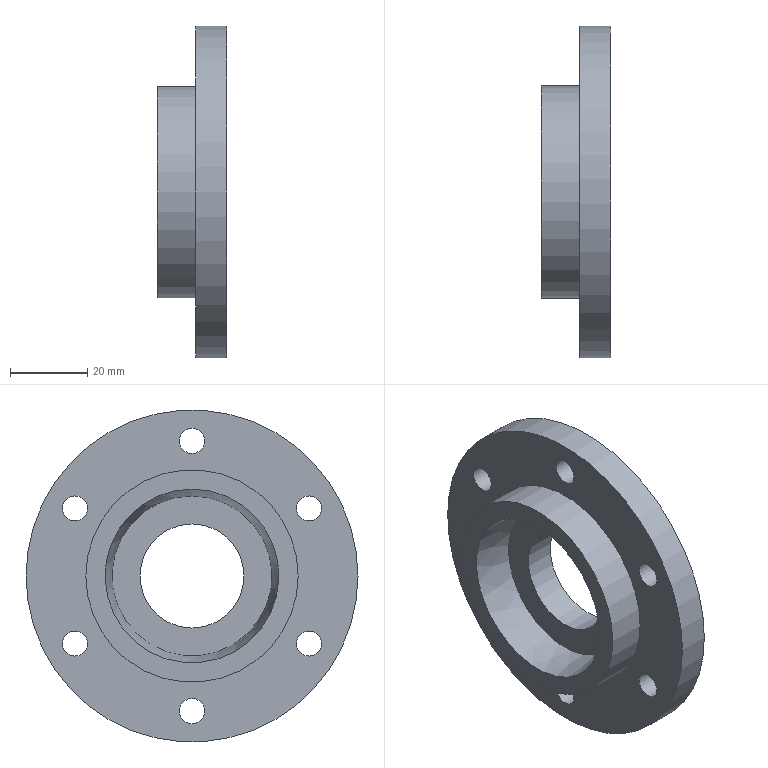Component | NX | XIAODUANTOUGAI | 1 solid | 14 faces | volume 49365 mm3 | cylinder 9 | plane 4 | cone 1 | commonest cylinder face diameters 6.5 x6 86 x1 55 x1 27 x1